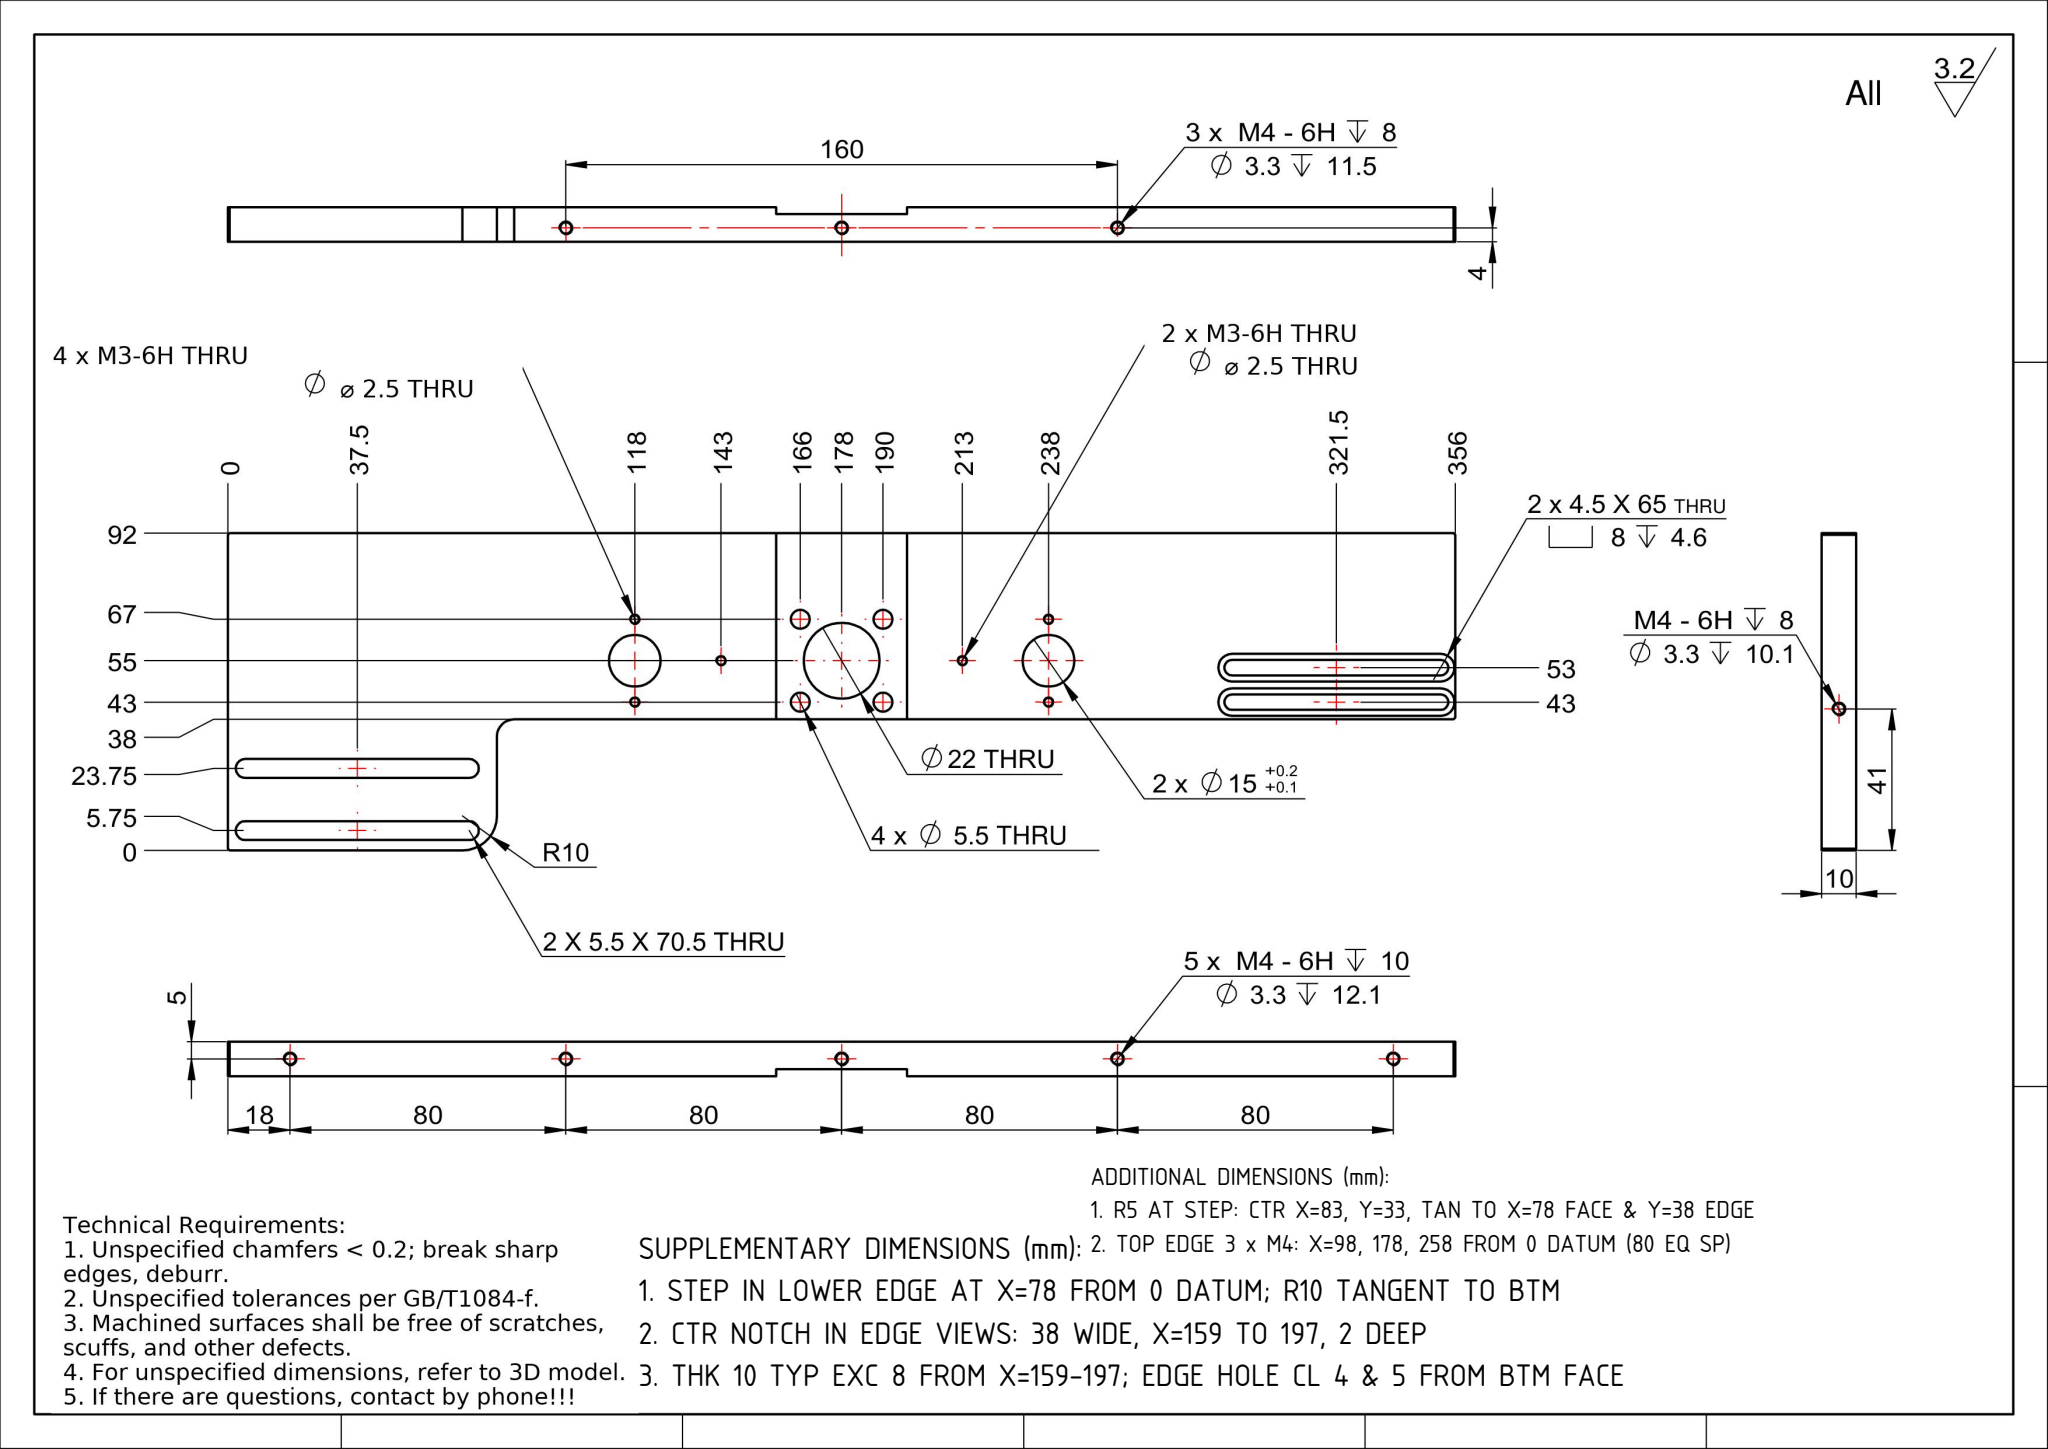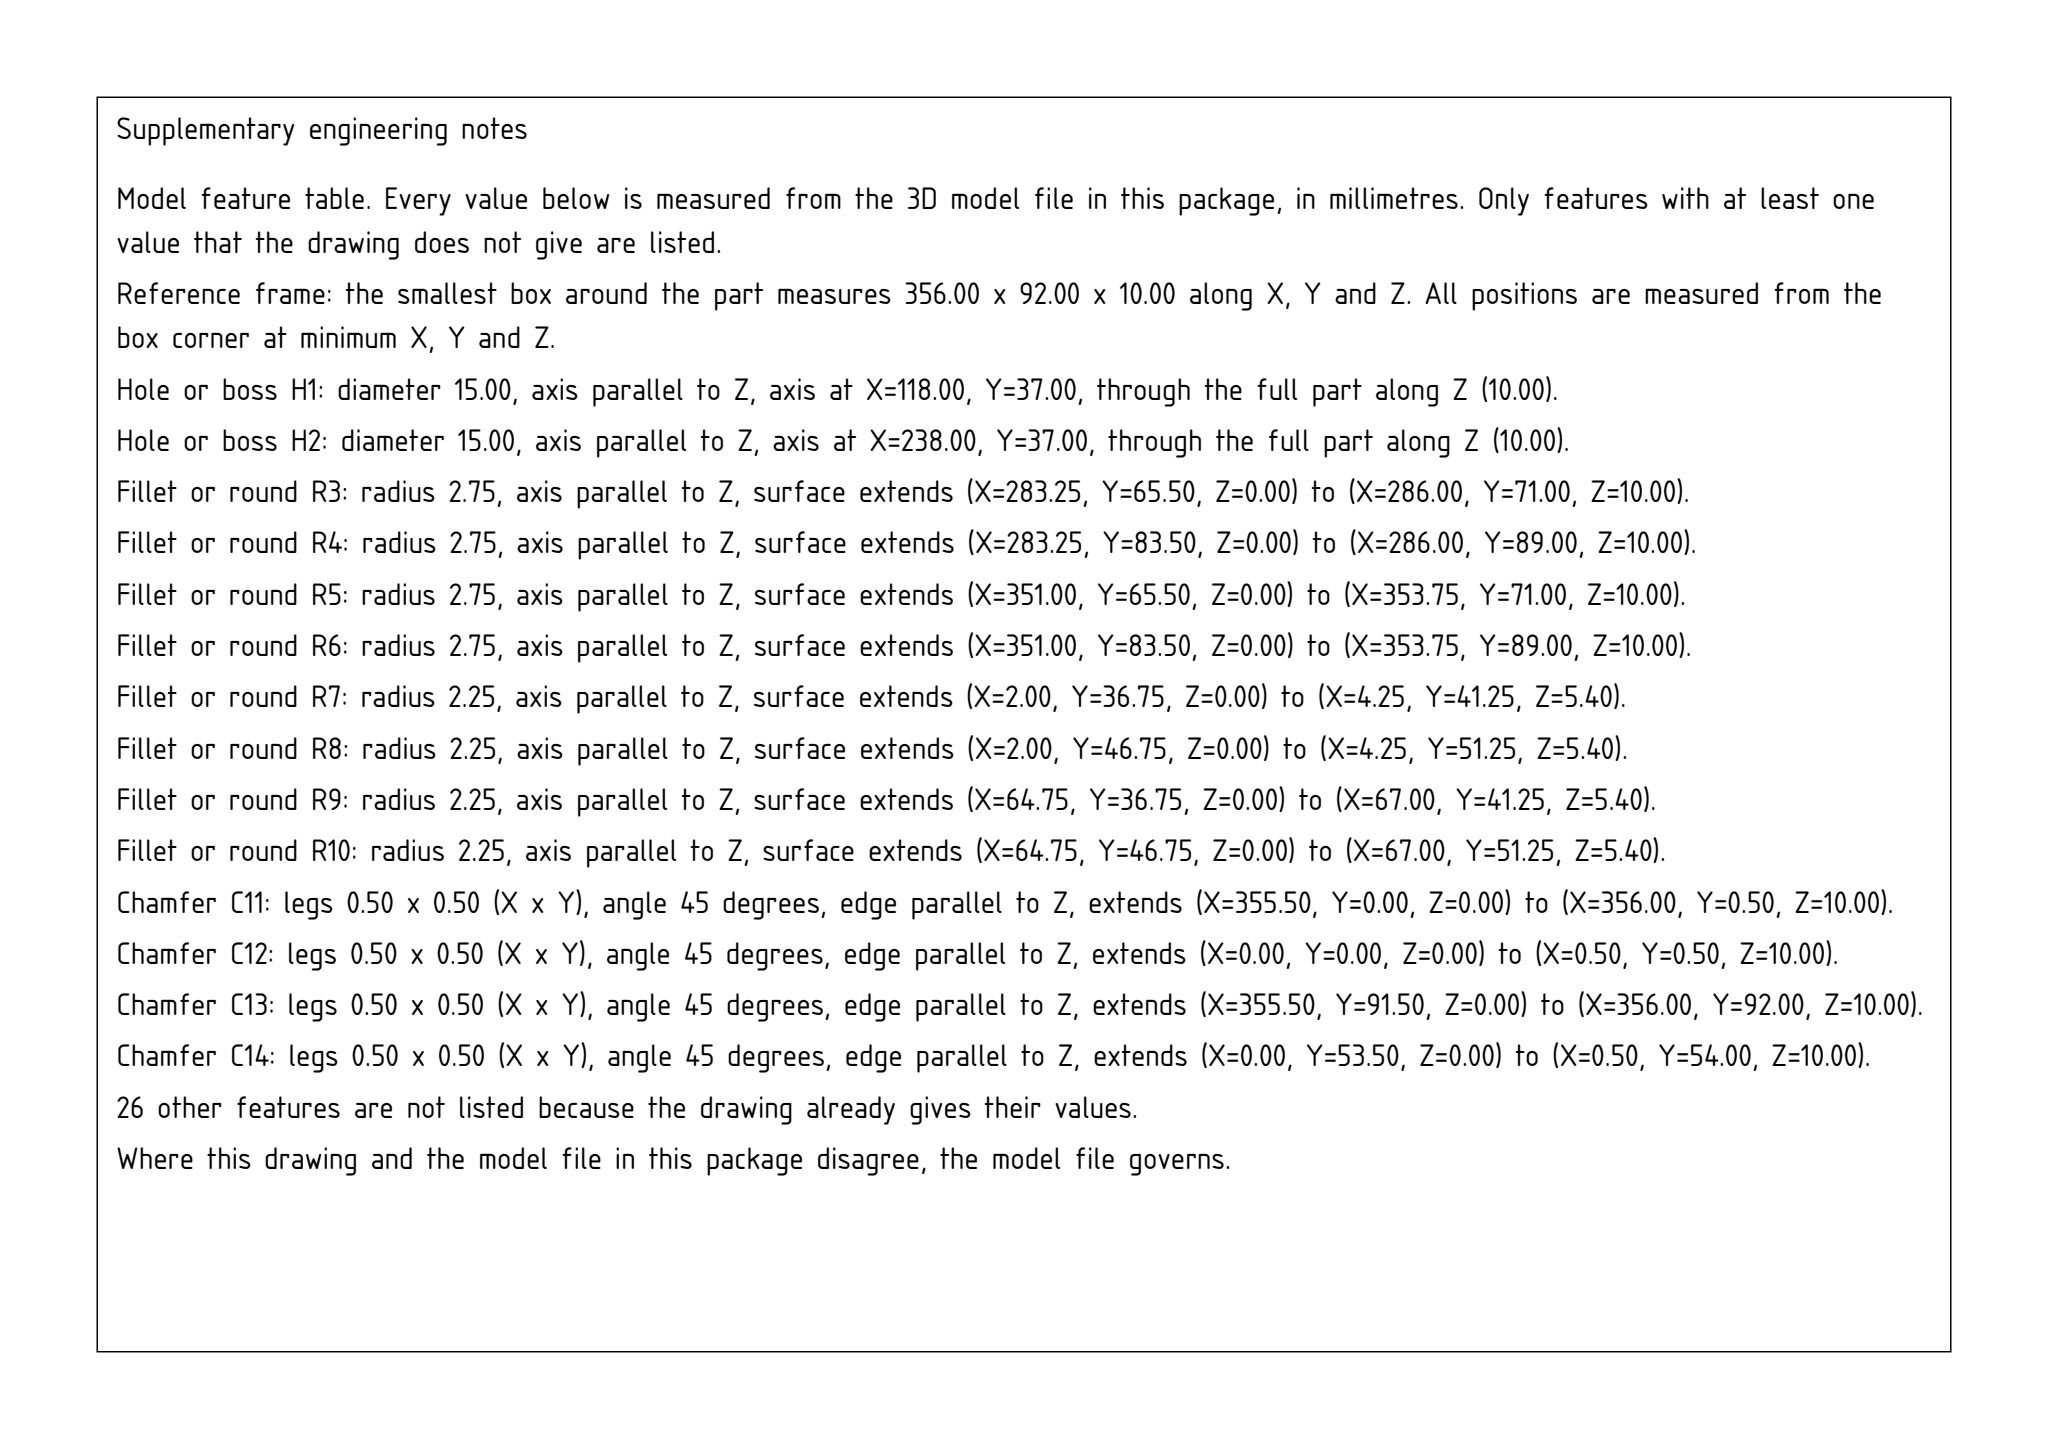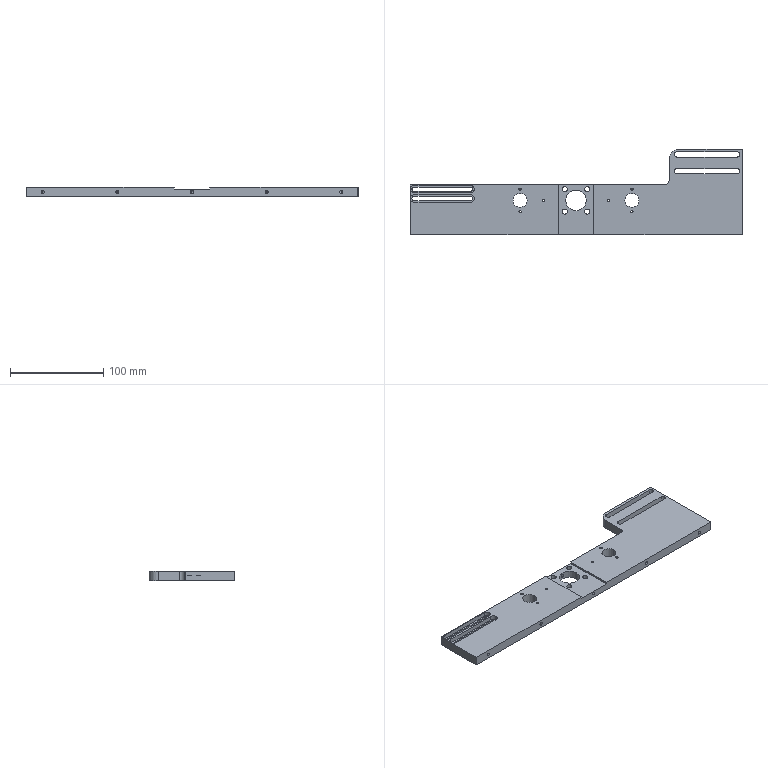Part | SolidWorks | mm | 1 solid | 110 faces | box 356 x 92 x 10 mm | volume 193453 mm3 | cylinder 64 | plane 30 | cone 16 | commonest cylinder face diameters 3.3 x18 5.5 x14 2.5 x12 8 x6 4.5 x6 15 x4 22 x2 20 x1